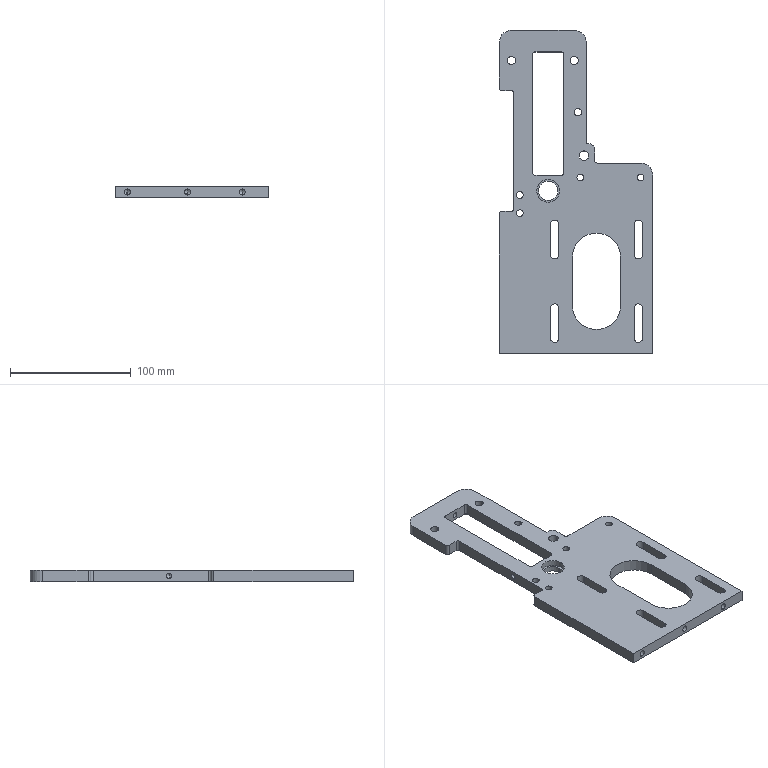Component | SolidWorks | FrameLeftPlate.1-1 | 1 solid | 90 faces | box 127 x 268 x 9.4 mm | volume 186461 mm3 | cylinder 53 | plane 29 | cone 8 | commonest cylinder face diameters 4 x9 5.5 x8 7 x8 5 x6 4.2 x4 6.8 x4 20 x3 16 x2
build123d program:
from build123d import *

# Parameters (mm, degrees)
SKETCH1_R                      = 4
SKETCH1_R_2                    = 9.5
SKETCH1_R_3                    = 3
BOSS_EXTRUDE1_DEPTH            = 9.4
M8_TAPPED_HOLE1_D              = 6.8
M8_TAPPED_HOLE1_DEPTH          = 19.75
M8_TAPPED_HOLE1_TIP            = 2.043
F_5_5_5_5_DIAMETER_HOLE1_D     = 5.5
F_5_5_5_5_DIAMETER_HOLE1_DEPTH = 10
F_5_5_5_5_DIAMETER_HOLE1_TIP   = 1.652
F_5_5_5_5_DIAMETER_HOLE2_D     = 5.5
F_5_5_5_5_DIAMETER_HOLE2_DEPTH = 10
F_5_5_5_5_DIAMETER_HOLE2_TIP   = 1.652
M5_TAPPED_HOLE3_D              = 4.2
M5_TAPPED_HOLE3_DEPTH          = 12.4
M5_TAPPED_HOLE3_TIP            = 1.262
CUT_EXTRUDE1_DEPTH             = 10
M5_TAPPED_HOLE4_D              = 4.2
M5_TAPPED_HOLE4_DEPTH          = 20
M5_TAPPED_HOLE4_TIP            = 1.262
M6_TAPPED_HOLE1_D              = 5
M6_TAPPED_HOLE1_DEPTH          = 15
M6_TAPPED_HOLE1_TIP            = 1.502
BOSS_EXTRUDE3_START            = -9.4
SKETCH16_R                     = 9.5
SKETCH16_R_2                   = 8
BOSS_EXTRUDE3_DEPTH            = 4.4


with BuildPart() as part:
    # Sketch1 → Boss-Extrude1 (new body)
    with BuildSketch(Plane.XY):
        with BuildLine():
            Line((81, 158), (117, 158))
            ThreePointArc((117, 158), (124.071, 155.071), (127, 148))
            Line((127, 148), (127, 0))
            Line((127, 0), (0, 0))
            Line((0, 0), (0, 116))
            ThreePointArc((0, 116), (0.5858, 117.414), (2, 118))
            Line((2, 118), (10, 118))
            ThreePointArc((10, 118), (11.414, 118.586), (12, 120))
            Line((12, 120), (12, 216))
            ThreePointArc((12, 216), (11.414, 217.414), (10, 218))
            Line((10, 218), (2, 218))
            ThreePointArc((2, 218), (0.5858, 218.586), (0, 220))
            Line((0, 220), (0, 258))
            ThreePointArc((0, 258), (2.929, 265.071), (10, 268))
            Line((10, 268), (62, 268))
            ThreePointArc((62, 268), (69.071, 265.071), (72, 258))
            Line((72, 258), (72, 174))
            Line((72, 174), (74, 174))
            ThreePointArc((74, 174), (77.536, 172.536), (79, 169))
            Line((79, 169), (79, 160))
            ThreePointArc((79, 160), (79.586, 158.586), (81, 158))
        make_face()
        with Locations((70, 164)):
            Circle(SKETCH1_R, mode=Mode.SUBTRACT)
        with Locations((40.5, 135)):
            Circle(SKETCH1_R_2, mode=Mode.SUBTRACT)
        with Locations((65, 200)):
            Circle(SKETCH1_R_3, mode=Mode.SUBTRACT)
        with BuildLine():
            Line((29.5, 250), (51.5, 250))
            ThreePointArc((51.5, 250), (52.914, 249.414), (53.5, 248))
            Line((53.5, 248), (53.5, 150))
            ThreePointArc((53.5, 150), (52.914, 148.586), (51.5, 148))
            Line((51.5, 148), (29.5, 148))
            ThreePointArc((29.5, 148), (28.086, 148.586), (27.5, 150))
            Line((27.5, 150), (27.5, 248))
            ThreePointArc((27.5, 248), (28.086, 249.414), (29.5, 250))
        make_face(mode=Mode.SUBTRACT)
    extrude(amount=BOSS_EXTRUDE1_DEPTH)

    # M8 Tapped Hole1
    with Locations(Plane.XY.offset(9.4)):
        with Locations((62, 243), (10, 243)):
            Hole(M8_TAPPED_HOLE1_D / 2, depth=M8_TAPPED_HOLE1_DEPTH)
            with Locations((0, 0, -(M8_TAPPED_HOLE1_DEPTH + M8_TAPPED_HOLE1_TIP / 2))):  # 118° drill point
                Cone(0, M8_TAPPED_HOLE1_D / 2, M8_TAPPED_HOLE1_TIP, mode=Mode.SUBTRACT)

    # 5.5 _5.5_ Diameter Hole1
    with Locations(Plane.XY.offset(9.4)):
        with Locations((17, 131.5), (17, 116.5)):
            Hole(F_5_5_5_5_DIAMETER_HOLE1_D / 2, depth=F_5_5_5_5_DIAMETER_HOLE1_DEPTH)
            with Locations((0, 0, -(F_5_5_5_5_DIAMETER_HOLE1_DEPTH + F_5_5_5_5_DIAMETER_HOLE1_TIP / 2))):  # 118° drill point
                Cone(0, F_5_5_5_5_DIAMETER_HOLE1_D / 2, F_5_5_5_5_DIAMETER_HOLE1_TIP, mode=Mode.SUBTRACT)

    # 5.5 _5.5_ Diameter Hole2
    with Locations(Plane.XY.offset(9.4)):
        with Locations((117, 146), (67, 146)):
            Hole(F_5_5_5_5_DIAMETER_HOLE2_D / 2, depth=F_5_5_5_5_DIAMETER_HOLE2_DEPTH)
            with Locations((0, 0, -(F_5_5_5_5_DIAMETER_HOLE2_DEPTH + F_5_5_5_5_DIAMETER_HOLE2_TIP / 2))):  # 118° drill point
                Cone(0, F_5_5_5_5_DIAMETER_HOLE2_D / 2, F_5_5_5_5_DIAMETER_HOLE2_TIP, mode=Mode.SUBTRACT)

    # M5 Tapped Hole3
    with Locations(Plane.ZY.offset(-12)):
        with Locations((4.9, 153)):
            Hole(M5_TAPPED_HOLE3_D / 2, depth=M5_TAPPED_HOLE3_DEPTH)
            with Locations((0, 0, -(M5_TAPPED_HOLE3_DEPTH + M5_TAPPED_HOLE3_TIP / 2))):  # 118° drill point
                Cone(0, M5_TAPPED_HOLE3_D / 2, M5_TAPPED_HOLE3_TIP, mode=Mode.SUBTRACT)

    # Sketch10 → Cut-Extrude1 (cut)
    with BuildSketch(Plane.XY.offset(9.4)):
        with BuildLine():
            Line((49.35, 37.85), (49.35, 12.85))
            ThreePointArc((49.35, 12.85), (45.85, 9.35), (42.35, 12.85))
            Line((42.35, 12.85), (42.35, 37.85))
            ThreePointArc((42.35, 37.85), (45.85, 41.35), (49.35, 37.85))
        make_face()
        with BuildLine():
            Line((111.65, 12.85), (111.65, 37.85))
            ThreePointArc((111.65, 37.85), (115.15, 41.35), (118.65, 37.85))
            Line((118.65, 37.85), (118.65, 12.85))
            ThreePointArc((118.65, 12.85), (115.15, 9.35), (111.65, 12.85))
        make_face()
        with BuildLine():
            Line((118.65, 107.15), (118.65, 82.15))
            ThreePointArc((118.65, 82.15), (115.15, 78.65), (111.65, 82.15))
            Line((111.65, 82.15), (111.65, 107.15))
            ThreePointArc((111.65, 107.15), (115.15, 110.65), (118.65, 107.15))
        make_face()
        with BuildLine():
            Line((49.35, 107.15), (49.35, 82.15))
            ThreePointArc((49.35, 82.15), (45.85, 78.65), (42.35, 82.15))
            Line((42.35, 82.15), (42.35, 107.15))
            ThreePointArc((42.35, 107.15), (45.85, 110.65), (49.35, 107.15))
        make_face()
        with BuildLine():
            Line((100.5, 80), (100.5, 40))
            ThreePointArc((100.5, 40), (80.5, 20), (60.5, 40))
            Line((60.5, 40), (60.5, 80))
            ThreePointArc((60.5, 80), (80.5, 100), (100.5, 80))
        make_face()
    extrude(amount=-CUT_EXTRUDE1_DEPTH, mode=Mode.SUBTRACT)

    # M5 Tapped Hole4
    with Locations(Plane(origin=(0, 268, 0), x_dir=(-1, 0, 0), z_dir=(0, 1, 0))):
        with Locations((-40.5, 4.7)):
            Hole(M5_TAPPED_HOLE4_D / 2, depth=M5_TAPPED_HOLE4_DEPTH)
            with Locations((0, 0, -(M5_TAPPED_HOLE4_DEPTH + M5_TAPPED_HOLE4_TIP / 2))):  # 118° drill point
                Cone(0, M5_TAPPED_HOLE4_D / 2, M5_TAPPED_HOLE4_TIP, mode=Mode.SUBTRACT)

    # M6 Tapped Hole1
    with Locations(Plane.XZ):
        with Locations((10, 4.7), (60, 4.7), (105, 4.7)):
            Hole(M6_TAPPED_HOLE1_D / 2, depth=M6_TAPPED_HOLE1_DEPTH)
            with Locations((0, 0, -(M6_TAPPED_HOLE1_DEPTH + M6_TAPPED_HOLE1_TIP / 2))):  # 118° drill point
                Cone(0, M6_TAPPED_HOLE1_D / 2, M6_TAPPED_HOLE1_TIP, mode=Mode.SUBTRACT)

    # Sketch16 → Boss-Extrude3 (add)
    with BuildSketch(Plane.XY.offset(9.4).offset(BOSS_EXTRUDE3_START)):
        with Locations((40.5, 135)):
            Circle(SKETCH16_R)
        with Locations((40.5, 135)):
            Circle(SKETCH16_R_2, mode=Mode.SUBTRACT)
    extrude(amount=BOSS_EXTRUDE3_DEPTH)


solid = part.part

# Placed as in the assembly
solid = solid.moved(Location((0, 0, -79.4), (0, 0, 0)))